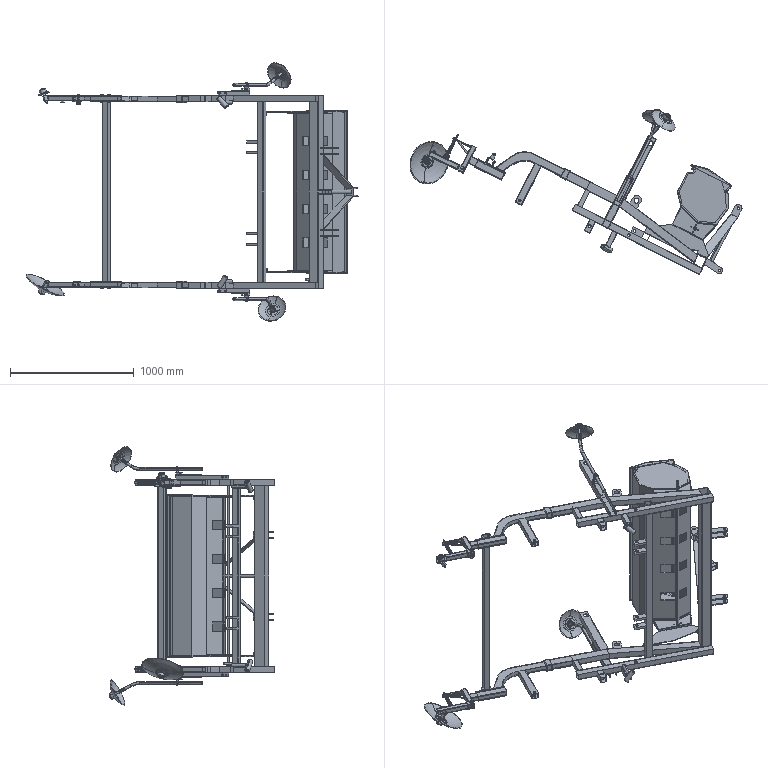Assembly | SolidWorks | mm | 102 component files | 111 solids | 2914 faces | box 2680.38 x 1339.53 x 2086.82 mm | volume 24526050 mm3 | plane 1099 | cylinder 917 | torus 468 | sphere 224 | cone 148 | spline 58 | commonest cylinder face diameters 20 x162 10 x114 8.5 x56 40 x50 8 x42 4 x40 12 x34 20.667 x32
Bill of materials:
AdjustmentEarPlate | 1 |  | U-shaped bent-sheet bracket: two parallel tapered flanges joined by a narrow web with rounded bends; each flange has a round hole near the web end.
Part24 | 2 |  | Combined profile: an open-ended thin-walled rectangular hollow tube with a round hollow tube of similar length lying along and joined to its top face.
Part26 | 2 |  | T-shaped part: a short thick-walled hollow cylinder with a smaller solid round rod sticking out at right angles from its side.
AttachedSoilDiskDiameter350 | 1 |  | Thin, shallow, concave dish-shaped disc with a central round hole and four smaller holes evenly spaced on a circle around it.
circlips for hole--type b gb | 4 |  | Flat split ring with a gap; the two ends form lugs that extend inward from the ring, each with a small round hole. The shape resembles an internal-style retaining ring.
circlips for shaft--type a large gb | 4 |  | Flat split ring with a narrow gap; the two ends form lugs that extend outward beyond the ring, each with a small round hole. The shape resembles an external-style retaining ring.
deep groove ball bearings gb | 8 |  | Ball-bearing-like ring assembly: an outer ring and an inner ring of equal width, with one row of spherical balls between them.
DustCover | 4 |  | Stepped annular ring: a wider, thin base flange with a smaller raised collar on top, a central through bore, and an open recess on the underside.
LargeAttachedSoilDiskAxis | 2 |  | Stepped cylindrical pin: a thin flat head, a long main shank, and a shorter reduced-diameter end section.
SoilDiskBearingHousing | 4 |  | Flanged sleeve: a hollow cylindrical boss on a thin circular flange that has four through holes evenly spaced around it.
AttachedSoilWheelVerticalAxis2 | 2 |  | T-shaped part: a short hollow cylindrical sleeve with a solid round rod sticking out at right angles from its side; the rod has a small cross hole near its free end.
FilmPressingSoilWheelBracket | 2 |  | T-shaped frame of thin-walled rectangular hollow tubes with a triangular gusset plate. The cross tube has a round hole, and a smaller telescoping-looking section with a hole extends from one end of a tube.
hex nuts with flange-fine pitch gb | 2 |  | Flanged hex nut-like body: hexagonal prism with a wider circular flange at one end and a plain central through-bore.
hexagon head bolts-full thread gb | 4 |  | Hex-head bolt-like part: hexagonal head on a plain cylindrical shank with a chamfered tip.
PressingFilmSoilPlateMovableFrame | 2 |  | Long arm with a rectangular cross-section: a cross-hole at one end, a forked (clevis-like) end with two parallel holed lugs at the other, and a pair of small parallel holed tabs sticking out from one side.
split pins | 2 |  | Split-pin-like part: two half-round legs side by side, joined by a looped eye at one end, with one leg longer than the other.
Spring3 | 2 |  | Helical coil spring made of round wire, with closely spaced end coils and evenly spaced open coils between them.
TieRod2 | 2 |  | Long cylindrical rod with a flat eye tab at one end and a circular collar near that end.
Part11 | 2 |  | Straight square or rectangular bar with a small holed tab sticking out sideways near one end.
Part5 | 2 |  | Short straight length of thin-walled rectangular tube, open at both ends.
Part5ConnectingSleeve | 2 |  | Short rectangular ring or sleeve with rounded outer edges, open through on one axis, with a raised rounded rib or seam across the faces.
Part6 | 2 |  | L-shaped frame made of two square or rectangular bars joined at roughly 90 degrees, with a through-hole near the free end of one arm.
Part7 | 2 |  | Straight length of thin-walled square or rectangular tube with open ends.
Part8 | 2 |  | Long slender square or rectangular tube with a single small round through-hole away from the ends.
PartFrameCorner | 2 |  | Welded-looking frame made of hollow rectangular tube: one long straight member with a smooth radiused bend at one end, plus a straight branch tube that joins it at an angle, forming a lambda/Y-like shape.
GB_T5781-2000[HexHeadBoltFullThreadGradeCM8_20] | 2 |  | Hex-head bolt-like part: a hexagonal head with a plain cylindrical shank coming out of one face. The shank has a chamfered free end, and there is a raised round collar/washer face between the head and the shank.
GB_T6174-2000[HexThinNutNoChamferM8] | 2 |  | Thin hexagonal nut-like part: a flat hex prism with one centred round through-hole, and chamfered corners on both faces.
Part10 | 1 |  | Straight length of hollow square tube with plain square-cut ends.
Part13 | 1 |  | Long hollow square tube with two pairs of thin parallel plate tabs sticking out from one side, one pair near each end. Each tab extends beyond the tube profile and has a round hole.
Part15 | 4 |  | Flat plate link with one rounded end that has a through hole; the plate widens toward the opposite, straight-cut end, which has a small corner chamfer.
Part17 | 1 |  | Thin flat plate with an irregular polygon outline and short bent flanges or lips along some edges, all turned to one side (downward in the side views).
Part18 | 1 |  | Thin flat plate with an irregular polygon outline and short flanges along some edges that point the opposite way from unnamed part (upward in the side views).
Part19 | 1 |  | Very slender solid round rod or pin with a constant diameter; the ends appear rounded or domed.
Part21 | 1 |  | Straight-cut spur gear with about 16 teeth, a central round bore and a cylindrical hub boss on one face.
Part28 | 2 |  | Short piece of hollow rectangular tube with open ends and one round through hole in a broad face.
Part40 | 1 |  | Straight length of hollow square tube with a relatively thick wall and plain ends.
PartThree | 4 |  | Flat plate with a constant thickness. One side has a wide rectangular notch that leaves two arms; the opposite side has two concave quarter-circle cutouts at its corners, leaving a narrower tongue.
AttachedSoilDisk | 2 |  | Thin dished (concave) circular disc with a flat central area that has a central round hole and four smaller holes evenly spaced around it.
AttachedSoilDiskAxis | 2 |  | Headed pin or bolt-like part: a thin, wide round head, a smooth cylindrical shank with a visible line around it partway along, and a grooved end section that looks threaded.
FilmBracketTube | 2 |  | Long, narrow formed sheet-metal channel (U- or hat-shaped cross-section), with a round hole near one end and a notch plus a bent hook or clip at the other end.
ScribingPlateFixedSleeve | 2 |  | Cylindrical sleeve that passes through a flat plate tab. The sleeve sticks out on both sides of the tab, and the tab has a stepped (L-shaped) top edge.
ScribingPlateMovableTube | 2 |  | Thin-walled round tube with one smooth bend near one end: a long straight leg and a short angled leg.
SeedBoxLidModification | 1 |  | Irregular polygonal plate with small notched tabs on one edge and a small hole pattern: a central hole with four smaller holes around it. The plate has a thicker region with raised edge walls or lips along part of its outline.
SeedBoxLidModificationOtherSide | 1 |  | Irregular polygonal flat plate with notched tabs on one edge, a central hole with four smaller holes around it, and one small hole near a tab. A region near one edge appears thicker.
SeedBoxModification | 1 |  | Long, open, roughly octagonal formed sheet-metal profile with hooked or stepped lips at both open edges, a row of rectangular slots along one face, and a small hole near one lip.
SeedBoxTopCover | 1 |  | Long, tapered, plate-like bracket or arm: a wide body that narrows toward a rounded lug with a round hole, plus a small stepped tab near the lug. One edge appears to have a narrow formed flange or lip.
TriangularHanger | 1 |  | V-shaped bracket made from two straight bars that meet at a vertex. At the vertex are a block with a hole and two parallel lugs with holes, in a clevis-like arrangement. The far ends of the bars are cut at an angle.
WeldedEarPlate | 1 |  | Flat tab: a rectangular block with one fully rounded end and one round through-hole centered on that rounded end. The opposite end is square.
WeldedPipe | 1 |  | Straight thin-walled round tube with plain square-cut ends.
Mates:
1. distance | Part15-4 face at (342.079, -1149.629, 1462.971) dir (0, 0, 1) | Part15-3 face at (342.079, -1149.629, 1502.971) dir (0, 0, -1)
2. coincident | AdjustmentEarPlate-1 face at (401.748, -1119.255, 1792.971) dir (0.4521, 0.892, 0) | WeldedPipe-1 edge at (366.069, -1101.171, 1812.971) dir (0.4521, 0.892, 0) r 16
3. concentric | TriangularHanger-1 edge at (550.526, -737.249, 1812.971) dir (0.4521, 0.892, 0) r 16 | WeldedPipe-1 edge at (551.43, -735.465, 1812.971) dir (0.4521, 0.892, 0) r 13
4. coincident | Part18-1 face at (350.003, -960.479, 1167.971) dir (0.4521, 0.892, 0) | SeedBoxAssemblyModified-1/SeedBoxLidModification-2 face at (47.001, -806.9, 1182.971) dir (-0.4521, -0.892, 0)
5. coincident | Part18-1 face at (298.812, -1061.476, 1162.971) dir (0, 0, -1) | SeedBoxAssemblyModified-1/SeedBoxLidModification-2 face at (240.361, -400.339, 1162.971) dir (0, 0, -1)
6. coincident | Part17-1 face at (45.644, -809.576, 2457.971) dir (-0.892, 0.4521, 0) | SeedBoxAssemblyModified-1/SeedBoxLidModificationOtherSide-1 face at (119.337, -664.185, 2442.971) dir (-0.892, 0.4521, 0)
7. coincident | SeedBoxAssemblyModified-1/SeedBoxLidModification-2 face at (214.293, -342.706, 1166.971) dir (0.4521, 0.892, 0) | SeedBoxTopCover-1 face at (196.453, -333.664, 1157.971) dir (-0.4521, -0.892, 0)
8. distance | SeedBoxAssemblyModified-1/SeedBoxModification-2 face at (526.481, -500.941, 2456.971) dir (0.892, -0.4521, 0) | SeedBoxTopCover-1 face at (526.481, -500.941, 1157.971) dir (0.892, -0.4521, 0)
9. concentric | SeedBoxTopCover-1 edge at (483.916, -540.681, 2467.971) dir (0, 0, 1) r 5 | GB_T5781-2000[HexHeadBoltFullThreadGradeCM8_20]-2 edge at (483.916, -540.681, 2448.971) dir (0, 0, 1) r 4
10. concentric | GB_T5781-2000[HexHeadBoltFullThreadGradeCM8_20]-1 edge at (483.792, -540.614, 1176.971) dir (0, 0, -1) r 4 | GB_T6174-2000[HexThinNutNoChamferM8]-1 edge at (483.792, -540.614, 1168.971) dir (0, 0, 1) r 4
11. concentric | GB_T5781-2000[HexHeadBoltFullThreadGradeCM8_20]-2 edge at (483.916, -540.681, 2448.971) dir (0, 0, 1) r 4 | GB_T6174-2000[HexThinNutNoChamferM8]-2 edge at (483.916, -540.681, 2456.971) dir (0, 0, 1) r 4
12. coincident | SeedBoxAssemblyModified-1/SeedBoxModification-2 face at (240.361, -400.339, 2456.971) dir (0, 0, -1) | GB_T6174-2000[HexThinNutNoChamferM8]-2 face at (477.416, -529.423, 2456.971) dir (0, 0, 1)
13. parallel | SeedBoxAssemblyModified-1/SeedBoxModification-2 face at (526.481, -500.941, 2456.971) dir (0.892, -0.4521, 0) | SeedBoxTopCover-1 face at (526.481, -500.941, 1157.971) dir (0.892, -0.4521, 0)
14. coincident | SeedBoxAssemblyModified-1/SeedBoxLidModification-2 face at (240.361, -400.339, 1162.971) dir (0, 0, -1) | SeedBoxTopCover-1 face at (466.915, -496.983, 1162.971) dir (0, 0, 1)
15. distance | GB_T6174-2000[HexThinNutNoChamferM8]-1 face at (477.292, -529.356, 1172.971) dir (0, 0, 1) | GB_T5781-2000[HexHeadBoltFullThreadGradeCM8_20]-1 face at (483.792, -540.614, 1177.971) dir (0, 0, 1)
16. distance | SeedBoxAssemblyModified-1/SeedBoxModification-2 face at (240.361, -400.339, 1168.971) dir (0, 0, 1) | GB_T6174-2000[HexThinNutNoChamferM8]-1 face at (477.292, -529.356, 1172.971) dir (0, 0, 1)
17. concentric | SeedBoxAssemblyModified-1/SeedBoxLidModification-2 edge at (483.792, -540.614, 1162.971) dir (0, 0, 1) r 4 | GB_T5781-2000[HexHeadBoltFullThreadGradeCM8_20]-1 edge at (483.792, -540.614, 1177.971) dir (0, 0, 1) r 3
18. concentric | GB_T5781-2000[HexHeadBoltFullThreadGradeCM8_20]-1 edge at (483.792, -540.614, 1176.971) dir (0, 0, -1) r 4 | GB_T6174-2000[HexThinNutNoChamferM8]-1 edge at (483.792, -540.614, 1172.971) dir (0, 0, 1) r 4
19. parallel | SeedBoxAssemblyModified-1/SeedBoxModification-2 face at (240.361, -400.339, 2456.971) dir (0, 0, -1) | GB_T6174-2000[HexThinNutNoChamferM8]-2 face at (477.416, -529.423, 2452.971) dir (0, 0, -1)
20. concentric | GB_T5781-2000[HexHeadBoltFullThreadGradeCM8_20]-2 edge at (483.916, -540.681, 2448.971) dir (0, 0, 1) r 4 | GB_T6174-2000[HexThinNutNoChamferM8]-2 edge at (483.916, -540.681, 2452.971) dir (0, 0, 1) r 4
21. distance | GB_T5781-2000[HexHeadBoltFullThreadGradeCM8_20]-2 face at (483.916, -540.681, 2447.971) dir (0, 0, -1) | GB_T6174-2000[HexThinNutNoChamferM8]-2 face at (477.416, -529.423, 2452.971) dir (0, 0, -1)
22. parallel | SeedBoxAssemblyModified-1/SeedBoxModification-2 face at (240.361, -400.339, 1168.971) dir (0, 0, 1) | GB_T5781-2000[HexHeadBoltFullThreadGradeCM8_20]-1 face at (483.792, -540.614, 1177.971) dir (0, 0, 1)
23. parallel | SeedBoxAssemblyModified-1/SeedBoxModification-2 face at (240.361, -400.339, 1168.971) dir (0, 0, 1) | GB_T5781-2000[HexHeadBoltFullThreadGradeCM8_20]-1 face at (483.792, -540.614, 1177.971) dir (0, 0, 1)
24. concentric | SeedBoxAssemblyModified-1/SeedBoxLidModificationOtherSide-1 edge at (231.081, -840.363, 2462.971) dir (0, 0, 1) r 13 | Part19-1 edge at (231.081, -840.363, 1045.971) dir (0, 0, 1) r 8.5
25. distance | Part19-1 face at (231.081, -840.363, 2582.971) dir (0, 0, 1) | SeedBoxAssemblyModified-1/SeedBoxLidModificationOtherSide-1 face at (240.361, -400.339, 2462.971) dir (0, 0, 1)
26. concentric | Part19-1 edge at (231.081, -840.363, 1045.971) dir (0, 0, 1) r 8.5 | Part21-2 edge at (231.081, -840.363, 1077.971) dir (0, 0, 1) r 16
27. distance | SeedBoxAssemblyModified-1/SeedBoxLidModification-2 face at (240.361, -400.339, 1162.971) dir (0, 0, -1) | Part21-2 face at (231.081, -840.363, 1097.971) dir (0, 0, -1)
28. coincident | Part17-1 face at (296.751, -933.488, 2457.971) dir (0.4521, 0.892, 0) | SeedBoxAssemblyModified-1/SeedBoxLidModificationOtherSide-1 face at (47.001, -806.9, 2442.971) dir (-0.4521, -0.892, 0)
29. coincident | Part17-1 face at (250.113, -1042.398, 2462.971) dir (0, 0, 1) | SeedBoxAssemblyModified-1/SeedBoxLidModificationOtherSide-1 face at (240.361, -400.339, 2462.971) dir (0, 0, 1)
30. coincident | FrameAssemblyDrawing11111-1/Part5-1 face at (-1544.877, -342.73, 1086.971) dir (-0.892, 0.4521, 0) | FrameAssemblyDrawing11111-Copy-1/Part5-1 face at (-1544.877, -342.73, 2590.971) dir (-0.892, 0.4521, 0)
31. parallel | FrameAssemblyDrawing11111-1/PartFrameCorner-1 face at (-1140.963, -396.106, 1080.971) dir (0, 0, 1) | FrameAssemblyDrawing11111-Copy-1/PartFrameCorner-1 face at (-1140.963, -396.106, 2544.971) dir (0, 0, -1)
32. coincident | FrameAssemblyDrawing11111-1/Part5-1 face at (-1543.521, -340.054, 1086.971) dir (0.4521, 0.892, 0) | PressingFilmSoilMechanism2-2/FilmPressingSoilWheelBracket-1 face at (-1329.449, -448.558, 1078.971) dir (-0.4521, -0.892, 0)
33. coincident | FrameAssemblyDrawing11111-1/Part5-1 face at (-1495.399, -380.35, 1083.971) dir (0, 0, -1) | PressingFilmSoilMechanism2-2/FilmPressingSoilWheelBracket-1 face at (-1327.189, -444.098, 1083.971) dir (0, 0, 1)
34. coincident | FrameAssemblyDrawing11111-1/Part5-1 face at (-1299.158, -388.796, 1086.971) dir (0.892, -0.4521, 0) | PressingFilmSoilMechanism2-2/FilmPressingSoilWheelBracket-1 face at (-1327.189, -444.098, 1048.971) dir (0.892, -0.4521, 0)
35. concentric | PressingFilmSoilMechanism2-2/AttachedSoilWheelVerticalAxis2-1 edge at (-1920.715, -303.338, 1046.651) dir (0.4522, -0.2133, 0.866) r 16 | AttachedSoilDiskDiameter350-2 edge at (-1930.212, -298.858, 1028.464) dir (-0.4522, 0.2133, -0.866) r 15
36. distance | AttachedSoilDiskDiameter350-2 face at (-1915.4, -246.677, 1037.046) dir (0.4522, -0.2133, 0.866) | PressingFilmSoilMechanism2-2/AttachedSoilWheelVerticalAxis2-1 face at (-1902.626, -311.87, 1081.292) dir (0.4522, -0.2133, 0.866)
37. coincident | FrameAssemblyDrawing11111-Copy-1/Part5-1 face at (-1543.521, -340.054, 2590.971) dir (0.4521, 0.892, 0) | FilmPressingSoilCoveringMechanism2Reverse-2/FilmPressingSoilWheelBracket-1 face at (-1329.449, -448.558, 2582.971) dir (-0.4521, -0.892, 0)
38. coincident | FrameAssemblyDrawing11111-Copy-1/Part5-1 face at (-1495.399, -380.35, 2587.971) dir (0, 0, -1) | FilmPressingSoilCoveringMechanism2Reverse-2/FilmPressingSoilWheelBracket-1 face at (-1327.189, -444.098, 2587.971) dir (0, 0, 1)
39. coincident | FrameAssemblyDrawing11111-Copy-1/Part5-1 face at (-1299.158, -388.796, 2590.971) dir (0.892, -0.4521, 0) | FilmPressingSoilCoveringMechanism2Reverse-2/FilmPressingSoilWheelBracket-1 face at (-1327.189, -444.098, 2552.971) dir (0.892, -0.4521, 0)
40. coincident | FrameAssemblyDrawing11111-Copy-1/Part5-1 face at (-1513.23, -280.292, 2590.971) dir (0.4521, 0.892, 0) | Part40-2 face at (-1406.194, -334.544, 1040.971) dir (-0.4521, -0.892, 0)
41. coincident | FrameAssemblyDrawing11111-Copy-1/Part5-1 face at (-1495.399, -380.35, 2590.971) dir (0, 0, 1) | Part40-2 face at (-1396.758, -291.07, 2590.971) dir (0, 0, 1)
42. distance | Part40-2 face at (-1450.793, -311.939, 1040.971) dir (-0.892, 0.4521, 0) | FrameAssemblyDrawing11111-Copy-1/Part5-1 face at (-1544.877, -342.73, 2590.971) dir (-0.892, 0.4521, 0)
43. distance | SeedBoxAssemblyModified-1/SeedBoxLidModification-2 face at (119.337, -664.185, 1182.971) dir (-0.892, 0.4521, 0) | Part18-1 face at (45.644, -809.576, 1182.971) dir (-0.892, 0.4521, 0)
44. coincident | FrameAssemblyDrawing11111-1/Part8-1 face at (-697.013, -707.415, 1035.971) dir (0, 0, -1) | Part10-1 face at (259.033, -1046.919, 1035.971) dir (0, 0, -1)
45. coincident | FrameAssemblyDrawing11111-1/Part8-1 face at (-733.735, -644.627, 1085.971) dir (0.4521, 0.892, 0) | Part10-1 face at (218.344, -1127.196, 1035.971) dir (-0.4521, -0.892, 0)
46. coincident | FrameAssemblyDrawing11111-1/Part11-2 face at (224.515, -1115.02, 1085.971) dir (0.892, -0.4521, 0) | Part10-1 face at (228.832, -1106.504, 1097.113) dir (-0.892, 0.4521, 0)
47. parallel | FrameAssemblyDrawing11111-Copy-1/Part8-1 face at (-697.013, -707.415, 2589.971) dir (0, 0, 1) | Part10-1 face at (259.033, -1046.919, 2589.971) dir (0, 0, 1)
48. coincident | Part17-1 face at (296.552, -1065.936, 2432.971) dir (-0.4521, -0.892, 0) | Part10-1 face at (259.033, -1046.919, 1035.971) dir (0.4521, 0.892, 0)
49. parallel | Part17-1 face at (250.113, -1042.398, 2462.971) dir (0, 0, 1) | FrameAssemblyDrawing11111-Copy-1/Part8-1 face at (-697.013, -707.415, 2589.971) dir (0, 0, 1)
50. coincident | Part17-1 face at (330.39, -1083.087, 2462.971) dir (0.892, -0.4521, 0) | Part10-1 face at (300.189, -1142.672, 1097.113) dir (0.892, -0.4521, 0)
51. distance | Part18-1 face at (298.812, -1061.476, 1162.971) dir (0, 0, -1) | FrameAssemblyDrawing11111-1/Part11-2 face at (-325.695, -673.671, 1085.971) dir (0, 0, 1)
52. parallel | Part17-1 face at (250.113, -1042.398, 2462.971) dir (0, 0, 1) | FrameAssemblyDrawing11111-Copy-1/Part11-2 face at (-325.695, -673.671, 2539.971) dir (0, 0, -1)
53. coincident | FrameAssemblyDrawing11111-Copy-1/Part8-1 face at (-697.013, -707.415, 2589.971) dir (0, 0, 1) | Part13-1 face at (-131.289, -893.926, 2589.971) dir (0, 0, 1)
54. coincident | FrameAssemblyDrawing11111-Copy-1/Part8-1 face at (-733.735, -644.627, 2589.971) dir (0.4521, 0.892, 0) | Part13-1 face at (-153.894, -938.524, 2589.971) dir (-0.4521, -0.892, 0)
55. coincident | Part17-1 face at (-174.531, -868.645, 2457.971) dir (-0.892, 0.4521, 0) | Part13-1 face at (-204.696, -928.158, 2528.83) dir (-0.892, 0.4521, 0)
56. parallel | Part17-1 face at (-129.933, -891.25, 2432.971) dir (0.892, -0.4521, 0) | Part13-1 face at (-160.098, -950.763, 2528.83) dir (0.892, -0.4521, 0)
57. coincident | FrameAssemblyDrawing11111-1/Part8-1 face at (-697.013, -707.415, 1035.971) dir (0, 0, -1) | Part13-1 face at (-131.289, -893.926, 1035.971) dir (0, 0, -1)
58. coincident | FrameAssemblyDrawing11111-1/Part8-1 face at (-733.735, -644.627, 1085.971) dir (0.4521, 0.892, 0) | Part13-1 face at (-153.894, -938.524, 2589.971) dir (-0.4521, -0.892, 0)
59. coincident | TriangularHanger-1 face at (259.033, -1046.919, 1512.971) dir (-0.4521, -0.892, 0) | Part10-1 face at (259.033, -1046.919, 1035.971) dir (0.4521, 0.892, 0)
60. distance | TriangularHanger-1 face at (259.033, -1046.919, 1452.971) dir (0, 0, -1) | Part10-1 face at (259.033, -1046.919, 1035.971) dir (0, 0, -1)
61. coincident | TriangularHanger-1 face at (334.007, -1075.951, 1337.971) dir (0.892, -0.4521, 0) | Part10-1 face at (300.189, -1142.672, 1097.113) dir (0.892, -0.4521, 0)
62. coincident | WeldedPipe-1 face at (366.069, -1101.171, 1812.971) dir (-0.4521, -0.892, 0) | Part10-1 face at (259.033, -1046.919, 1035.971) dir (0.4521, 0.892, 0)
63. coincident | AdjustmentEarPlate-1 face at (330.39, -1083.087, 1792.971) dir (-0.892, 0.4521, 0) | Part10-1 face at (300.189, -1142.672, 1097.113) dir (0.892, -0.4521, 0)
64. distance | AdjustmentEarPlate-1 face at (379.326, -1130.313, 1792.971) dir (0, 0, -1) | Part10-1 face at (259.033, -1046.919, 1035.971) dir (0, 0, -1)
65. distance | Part15-4 face at (342.079, -1149.629, 1452.971) dir (0, 0, -1) | Part10-1 face at (259.033, -1046.919, 1035.971) dir (0, 0, -1)
66. coincident | Part15-4 face at (305.946, -1131.315, 1462.971) dir (-0.892, 0.4521, 0) | Part10-1 face at (300.189, -1142.672, 1097.113) dir (0.892, -0.4521, 0)
67. coincident | Part15-4 face at (366.524, -1101.402, 1462.971) dir (0.4521, 0.892, 0) | Part10-1 face at (259.033, -1046.919, 1035.971) dir (0.4521, 0.892, 0)
68. coincident | Part15-3 face at (305.946, -1131.315, 1512.971) dir (-0.892, 0.4521, 0) | Part10-1 face at (300.189, -1142.672, 1097.113) dir (0.892, -0.4521, 0)
69. coincident | Part15-3 face at (366.524, -1101.402, 1512.971) dir (0.4521, 0.892, 0) | Part10-1 face at (259.033, -1046.919, 1035.971) dir (0.4521, 0.892, 0)
70. distance | Part15-2 face at (342.079, -1149.629, 2172.971) dir (0, 0, 1) | Part10-1 face at (259.033, -1046.919, 2589.971) dir (0, 0, 1)
71. coincident | Part15-2 face at (305.946, -1131.315, 2172.971) dir (-0.892, 0.4521, 0) | Part10-1 face at (300.189, -1142.672, 1097.113) dir (0.892, -0.4521, 0)
72. coincident | Part15-2 face at (366.524, -1101.402, 2172.971) dir (0.4521, 0.892, 0) | Part10-1 face at (259.033, -1046.919, 1035.971) dir (0.4521, 0.892, 0)
73. coincident | Part15-1 face at (305.946, -1131.315, 2122.971) dir (-0.892, 0.4521, 0) | Part10-1 face at (300.189, -1142.672, 1097.113) dir (0.892, -0.4521, 0)
74. coincident | Part15-1 face at (366.524, -1101.402, 2122.971) dir (0.4521, 0.892, 0) | Part10-1 face at (259.033, -1046.919, 1035.971) dir (0.4521, 0.892, 0)
75. distance | Part15-1 face at (342.079, -1149.629, 2122.971) dir (0, 0, 1) | Part15-2 face at (342.079, -1149.629, 2162.971) dir (0, 0, -1)
76. coincident | PartThree-2 face at (-1397.275, -339.065, 1040.971) dir (-0.4521, -0.892, 0) | FrameAssemblyDrawing11111-1/Part5-1 face at (-1513.23, -280.292, 1086.971) dir (0.4521, 0.892, 0)
77. coincident | PartThree-2 face at (-1404.056, -352.445, 1040.971) dir (0, 0, 1) | FrameAssemblyDrawing11111-1/Part5-1 face at (-1495.399, -380.35, 1040.971) dir (0, 0, -1)
78. coincident | PartThree-2 face at (-1404.942, -332.074, 1058.529) dir (-0.892, 0.4521, 0) | Part40-2 face at (-1406.194, -334.544, 1040.971) dir (0.892, -0.4521, 0)
79. coincident | PartThree-1 face at (-1459.712, -307.418, 1086.971) dir (-0.4521, -0.892, 0) | FrameAssemblyDrawing11111-1/Part5-1 face at (-1513.23, -280.292, 1086.971) dir (0.4521, 0.892, 0)
80. coincident | PartThree-1 face at (-1466.494, -320.798, 1086.971) dir (0, 0, -1) | FrameAssemblyDrawing11111-1/Part5-1 face at (-1495.399, -380.35, 1086.971) dir (0, 0, 1)
81. coincident | PartThree-1 face at (-1449.541, -309.469, 1069.414) dir (0.892, -0.4521, 0) | Part40-2 face at (-1450.793, -311.939, 1040.971) dir (-0.892, 0.4521, 0)
82. coincident | PartThree-3 face at (-1450.793, -311.939, 2544.971) dir (-0.4521, -0.892, 0) | FrameAssemblyDrawing11111-Copy-1/Part5-1 face at (-1513.23, -280.292, 2590.971) dir (0.4521, 0.892, 0)
83. coincident | PartThree-3 face at (-1457.574, -325.319, 2590.971) dir (0, 0, -1) | FrameAssemblyDrawing11111-Copy-1/Part5-1 face at (-1495.399, -380.35, 2590.971) dir (0, 0, 1)
84. coincident | PartThree-3 face at (-1449.541, -309.469, 2562.529) dir (0.892, -0.4521, 0) | Part40-2 face at (-1450.793, -311.939, 1040.971) dir (-0.892, 0.4521, 0)
85. coincident | PartThree-4 face at (-1406.194, -334.544, 2590.971) dir (-0.4521, -0.892, 0) | FrameAssemblyDrawing11111-Copy-1/Part5-1 face at (-1513.23, -280.292, 2590.971) dir (0.4521, 0.892, 0)
86. coincident | PartThree-4 face at (-1412.976, -347.924, 2544.971) dir (0, 0, 1) | FrameAssemblyDrawing11111-Copy-1/Part5-1 face at (-1495.399, -380.35, 2544.971) dir (0, 0, -1)
87. coincident | PartThree-4 face at (-1404.942, -332.074, 2573.414) dir (-0.892, 0.4521, 0) | Part40-2 face at (-1406.194, -334.544, 1040.971) dir (0.892, -0.4521, 0)
88. coincident | ScribingMechanismAssembly-2/FilmBracketTube-1 face at (-515.635, -816.834, 2624.971) dir (-0.4521, -0.892, 0) | FrameAssemblyDrawing11111-Copy-1/Part8-1 face at (-758.601, -693.686, 2589.971) dir (-0.4521, -0.892, 0)
89. coincident | ScribingMechanismAssembly-2/FilmBracketTube-1 face at (-312.19, -415.449, 2589.971) dir (0, 0, -1) | FrameAssemblyDrawing11111-Copy-1/Part8-1 face at (-697.013, -707.415, 2589.971) dir (0, 0, 1)
90. distance | ScribingMechanismAssembly-2/FilmBracketTube-1 face at (-263.132, -440.315, 2594.971) dir (0.892, -0.4521, 0) | Part10-1 face at (300.189, -1142.672, 1097.113) dir (0.892, -0.4521, 0)
91. coincident | ScribingMechanismAssembly-1/FilmBracketTube-1 face at (-471.037, -839.439, 1000.971) dir (-0.4521, -0.892, 0) | FrameAssemblyDrawing11111-1/Part8-1 face at (-758.601, -693.686, 1085.971) dir (-0.4521, -0.892, 0)
92. coincident | ScribingMechanismAssembly-1/FilmBracketTube-1 face at (-267.592, -438.054, 1035.971) dir (0, 0, 1) | FrameAssemblyDrawing11111-1/Part11-2 face at (-325.695, -673.671, 1035.971) dir (0, 0, -1)
93. distance | ScribingMechanismAssembly-1/FilmBracketTube-1 face at (-263.132, -440.315, 1030.971) dir (0.892, -0.4521, 0) | Part10-1 face at (300.189, -1142.672, 1097.113) dir (0.892, -0.4521, 0)
94. coincident | Assembly4-1/Part24-1 face at (-413.302, -868.703, 1089.08) dir (0.4521, 0.892, 0) | FrameAssemblyDrawing11111-1/Part8-1 face at (-758.601, -693.686, 1085.971) dir (-0.4521, -0.892, 0)
95. coincident | Assembly4-1/Part24-1 face at (-453.993, -993.824, 1035.971) dir (0, 0, -1) | FrameAssemblyDrawing11111-1/Part8-1 face at (-697.013, -707.415, 1035.971) dir (0, 0, -1)
96. distance | ScribingMechanismAssembly-1/FilmBracketTube-1 face at (-263.132, -440.315, 1030.971) dir (0.892, -0.4521, 0) | Assembly4-1/Part24-1 face at (-453.993, -993.824, 1075.971) dir (0.892, -0.4521, 0)
97. distance | AssemblyTillageDisc-1/Part24-1 face at (-453.993, -993.824, 2549.971) dir (0.892, -0.4521, 0) | ScribingMechanismAssembly-2/FilmBracketTube-1 face at (-263.132, -440.315, 2594.971) dir (0.892, -0.4521, 0)
98. coincident | AssemblyTillageDisc-1/Part24-1 face at (-490.156, -975.494, 2589.971) dir (0, 0, 1) | FrameAssemblyDrawing11111-Copy-1/Part8-1 face at (-697.013, -707.415, 2589.971) dir (0, 0, 1)
99. coincident | AssemblyTillageDisc-1/Part24-1 face at (-413.302, -868.703, 2536.863) dir (0.4521, 0.892, 0) | FrameAssemblyDrawing11111-Copy-1/Part8-1 face at (-758.601, -693.686, 2589.971) dir (-0.4521, -0.892, 0)
100. coincident | Part28-4 face at (-615.886, -766.022, 1085.971) dir (0.4521, 0.892, 0) | FrameAssemblyDrawing11111-1/Part8-1 face at (-758.601, -693.686, 1085.971) dir (-0.4521, -0.892, 0)
101. coincident | Part28-4 face at (-589.965, -818.378, 1035.971) dir (0, 0, -1) | FrameAssemblyDrawing11111-1/Part8-1 face at (-697.013, -707.415, 1035.971) dir (0, 0, -1)
102. coincident | Part28-3 face at (-615.886, -766.022, 2589.971) dir (0.4521, 0.892, 0) | FrameAssemblyDrawing11111-Copy-1/Part8-1 face at (-758.601, -693.686, 2589.971) dir (-0.4521, -0.892, 0)
103. coincident | Part28-3 face at (-589.965, -818.378, 2589.971) dir (0, 0, 1) | FrameAssemblyDrawing11111-Copy-1/Part8-1 face at (-697.013, -707.415, 2589.971) dir (0, 0, 1)
104. coincident | Part40-2 face at (-1383.589, -289.946, 1040.971) dir (0.4521, 0.892, 0) | WeldedEarPlate-5 face at (-1419.268, -271.862, 2550.971) dir (-0.4521, -0.892, 0)
105. distance | WeldedEarPlate-5 face at (-1390.065, -247.424, 2542.971) dir (0, 0, -1) | Part40-2 face at (-1396.758, -291.07, 2590.971) dir (0, 0, 1)
106. distance | Part40-2 face at (-1450.793, -311.939, 1040.971) dir (-0.892, 0.4521, 0) | WeldedEarPlate-5 face at (-1403.444, -240.643, 2550.971) dir (-0.892, 0.4521, 0)
107. distance | Part28-4 face at (-571.288, -788.627, 1085.971) dir (0.892, -0.4521, 0) | FrameAssemblyDrawing11111-1/Part8-1 face at (292.027, -1164.543, 1085.971) dir (0.892, -0.4521, 0)
108. distance | Part28-3 face at (-571.288, -788.627, 2589.971) dir (0.892, -0.4521, 0) | FrameAssemblyDrawing11111-Copy-1/Part8-1 face at (292.027, -1164.543, 2589.971) dir (0.892, -0.4521, 0)
109. concentric | Part24-1 face at (2.837, 36.367, 170) dir (0, -1, 0) r 15 | Part26-1 face at (2.837, -93.633, 170) dir (0, -1, 0) r 10
110. coincident | Part26-1 face at (2.837, -93.633, 170) dir (0, -1, 0) | Part24-1 face at (2.837, -93.633, 170) dir (0, -1, 0)
111. coincident | Part24-1 edge at (-24.743, 0.07636, 65) dir (0, 0, 1) r 10 | Part26-1 edge at (-24.743, 0.07636, 65) dir (0, 0, -1) r 10
112. concentric | FilmPressingSoilWheelBracket-1 face at (-20, -95, -170) dir (1, 0, 0) r 6 | PressingFilmSoilPlateMovableFrame-1 face at (25, -95, -170) dir (-1, 0, 0) r 6
113. coincident | FilmPressingSoilWheelBracket-1 face at (20, -120, -155) dir (1, 0, 0) | PressingFilmSoilPlateMovableFrame-1 face at (20, -115.929, -202.419) dir (-1, 0, 0)
114. concentric | PressingFilmSoilPlateMovableFrame-1 face at (0, 177.365, -442.841) dir (0, -0.9996, 0.02839) r 10 | AttachedSoilWheelVerticalAxis2-1 face at (0, -67.536, -435.887) dir (0, -0.9996, 0.02839) r 10
115. distance | AttachedSoilWheelVerticalAxis2-1 face at (0, -67.536, -435.887) dir (0, 0.9996, -0.02839) | PressingFilmSoilPlateMovableFrame-1 face at (-16, -83.24, -460.451) dir (0, 0.9996, -0.02839)
116. concentric | AttachedSoilWheelVerticalAxis2-1 face at (-18.794, -167.69, -439.886) dir (0.9397, 0.009709, 0.3419) r 10 | AttachedSoilDiskAssembly2-1/LargeAttachedSoilDiskAxis-1 face at (18.794, -167.302, -426.21) dir (-0.9397, -0.009709, -0.3419) r 10
117. coincident | AttachedSoilWheelVerticalAxis2-1 face at (18.794, -167.302, -426.21) dir (0.9397, 0.009709, 0.3419) | AttachedSoilDiskAssembly2-1/LargeAttachedSoilDiskAxis-1 face at (18.794, -167.302, -426.21) dir (0.9397, 0.009709, 0.3419)
118. angle | AttachedSoilWheelVerticalAxis2-1 face at (-18.794, -167.69, -439.886) dir (-0.9397, -0.009709, -0.3419) | PressingFilmSoilPlateMovableFrame-1 face at (20, -87.238, -460.337) dir (1, 0, 0)
119. concentric | AttachedSoilWheelVerticalAxis2-1 face at (-46.985, -79.017, -452.669) dir (0.9397, 0.009709, 0.3419) r 3 | split pins-1 face at (-9.794, -78.633, -439.138) dir (-0.9397, -0.009709, -0.3419) r 0.25
120. distance | split pins-1 face at (-12.613, -78.662, -440.164) dir (-0.9397, -0.009709, -0.3419) | AttachedSoilWheelVerticalAxis2-1 face at (0, -67.536, -435.887) dir (0, -0.9996, 0.02839) r 10
121. concentric | PressingFilmSoilPlateMovableFrame-1 face at (25, -95, -170) dir (-1, 0, 0) r 6 | hexagon head bolts-full thread gb-1 face at (10, -95, -170) dir (-1, 0, 0) r 4
122. coincident | PressingFilmSoilPlateMovableFrame-1 face at (-25, -114.424, -149.44) dir (-1, 0, 0) | hexagon head bolts-full thread gb-1 face at (-25, -95, -183) dir (1, 0, 0)
123. concentric | hexagon head bolts-full thread gb-1 face at (10, -95, -170) dir (-1, 0, 0) r 4 | hex nuts with flange-fine pitch gb-2 face at (25, -95, -170) dir (1, 0, 0) r 785.398
124. coincident | PressingFilmSoilPlateMovableFrame-1 face at (25, -115.929, -202.419) dir (1, 0, 0) | hex nuts with flange-fine pitch gb-2 face at (25, -110, -178.66) dir (-1, 0, 0)
125. concentric | PressingFilmSoilPlateMovableFrame-1 face at (-20, -62.057, -331) dir (1, 0, 0) r 5 | TieRod2-1 face at (27.5, -62.057, -331) dir (-1, 0, 0) r 5
126. distance | TieRod2-1 face at (2.5, -72.057, -321) dir (1, 0, 0) | PressingFilmSoilPlateMovableFrame-1 face at (5, -49.207, -318.86) dir (-1, 0, 0)
127. tangent | FilmPressingSoilWheelBracket-1 face at (0, -200, -330) dir (0, 1, 0) r 6 | TieRod2-1 face at (0, 137.943, -331) dir (0, -1, 0) r 5
128. concentric | TieRod2-1 face at (0, 137.943, -331) dir (0, -1, 0) r 5 | Spring3-1 sketch segment at (0, -22.057, -331) dir (0, 1, 0) r 10
129. coincident | TieRod2-1 face at (0, -22.057, -331) dir (0, 1, 0) | Spring3-1 face at (0, -22.057, -331) dir (0, -1, 0)
130. concentric | PressingFilmSoilPlateMovableFrame-1 face at (-20, -62.057, -331) dir (1, 0, 0) r 5 | hexagon head bolts-full thread gb-2 face at (25, -62.057, -331) dir (-1, 0, 0) r 4
131. coincident | PressingFilmSoilPlateMovableFrame-1 face at (-10, -49.207, -318.86) dir (-1, 0, 0) | hexagon head bolts-full thread gb-2 face at (-10, -62.057, -344) dir (1, 0, 0)
132. concentric | hexagon head bolts-full thread gb-2 face at (25, -62.057, -331) dir (-1, 0, 0) r 4 | hex nuts with flange-fine pitch gb-4 face at (10, -62.057, -331) dir (1, 0, 0) r 785.398
133. coincident | PressingFilmSoilPlateMovableFrame-1 face at (10, -49.207, -318.86) dir (1, 0, 0) | hex nuts with flange-fine pitch gb-4 face at (10, -77.057, -339.66) dir (-1, 0, 0)
134. concentric | SoilDiskBearingHousing-1 face at (72, 0, 0) dir (-1, 0, 0) r 23.5 | deep groove ball bearings gb-1 face at (59.289, 0, 0) dir (-1, 0, 0) r 13
135. coincident | SoilDiskBearingHousing-1 face at (72, 0, 0) dir (-1, 0, 0) | deep groove ball bearings gb-1 face at (72, 13, 0) dir (1, 0, 0)
136. concentric | SoilDiskBearingHousing-1 face at (72, 0, 0) dir (-1, 0, 0) r 23.5 | deep groove ball bearings gb-2 face at (51.289, 0, 0) dir (-1, 0, 0) r 13
137. coincident | deep groove ball bearings gb-1 face at (64, 13, 0) dir (-1, 0, 0) | deep groove ball bearings gb-2 face at (64, 13, 0) dir (1, 0, 0)
138. concentric | SoilDiskBearingHousing-1 face at (72, 0, 0) dir (-1, 0, 0) r 23.5 | circlips for hole--type b gb-1 face at (44, 0, 0) dir (-1, 0, 0) r 10.75
139. coincident | SoilDiskBearingHousing-1 face at (44, 0, 25.5) dir (-1, 0, 0) | circlips for hole--type b gb-1 face at (44, 0, 0) dir (1, 0, 0)
140. concentric | deep groove ball bearings gb-2 face at (53.029, 0, 0) dir (-1, 0, 0) r 5 | LargeAttachedSoilDiskAxis-1 face at (-21, 0, 0) dir (1, 0, 0) r 10
141. concentric | SoilDiskBearingHousing-1 face at (75, 0, 0) dir (-1, 0, 0) r 20 | DustCover-1 face at (77, 0, 0) dir (-1, 0, 0) r 20
142. coincident | SoilDiskBearingHousing-1 edge at (72, 0, 0) dir (-1, 0, 0) r 20 | DustCover-1 edge at (72, 0, 0) dir (1, 0, 0) r 20
143. concentric | LargeAttachedSoilDiskAxis-1 face at (-21, 0, 0) dir (1, 0, 0) r 10 | circlips for shaft--type a large gb-1 face at (43, 0, 0) dir (1, 0, 0) r 4.65
144. coincident | LargeAttachedSoilDiskAxis-1 face at (44, 2.228, -11.282) dir (-1, 0, 0) | circlips for shaft--type a large gb-1 face at (44, 0, 0) dir (1, 0, 0)
145. coincident | deep groove ball bearings gb-1 face at (72, 5, 0) dir (1, 0, 0) | LargeAttachedSoilDiskAxis-1 face at (72, 0, 0) dir (-1, 0, 0)
146. coincident | PartFrameCorner-1 face at (-461.187, -56.353, 753.41) dir (0, -1, 0) | Part5-1 face at (-612.187, -56.353, 759.41) dir (0, 1, 0)
147. distance | PartFrameCorner-1 edge at (-396.187, -56.353, 753.41) dir (0, 0, -1) | Part5-1 edge at (-372.187, -56.353, 759.41) dir (0, 0, -1)
148. coincident | PartFrameCorner-1 face at (-227.777, 8.647, 713.41) dir (0, 0, -1) | Part5-1 face at (-551.046, -137.54, 713.41) dir (0, 0, -1)
149. distance | Part5ConnectingSleeve-1 edge at (42.212, 186.082, 758.41) dir (0, 0, -1) | PartFrameCorner-1 edge at (-227.777, 183.647, 753.41) dir (0, 0, -1)
150. distance | PartFrameCorner-1 face at (-227.777, 8.647, 713.41) dir (0, 0, -1) | Part5ConnectingSleeve-1 face at (92.212, 191.082, 708.41) dir (0, 0, 1)
151. distance | Part5ConnectingSleeve-1 face at (92.212, 116.082, 703.41) dir (0, 1, 0) | PartFrameCorner-1 face at (-194.191, 118.515, 753.41) dir (0, -1, 0)
152. distance | PartFrameCorner-1 face at (-227.777, 8.647, 713.41) dir (0, 0, -1) | Part6-1 face at (114.746, 121.183, 710.41) dir (0, 0, 1)
153. distance | PartFrameCorner-1 face at (-227.777, 183.647, 753.41) dir (0, 1, 0) | Part6-1 face at (47.813, 184.082, 758.41) dir (0, -1, 0)
154. distance | Part6-1 face at (47.813, 186.082, 758.41) dir (-1, 0, 0) | Part5-1 face at (-372.187, -56.353, 759.41) dir (1, 0, 0)
155. distance | Part7-3 face at (267.813, 116.082, 758.41) dir (0, 0, 1) | Part6-1 face at (114.746, 121.183, 758.41) dir (0, 0, 1)
156. perpendicular | Part6-1 face at (47.813, 116.082, 758.41) dir (0, -1, 0) | Part7-3 face at (307.813, -78.46, 797.209) dir (1, 0, 0)
157. distance | Part7-3 face at (307.813, -78.46, 797.209) dir (1, 0, 0) | Part6-1 face at (577.813, 186.082, 758.41) dir (1, 0, 0)
158. distance | Part7-3 face at (267.813, -28.918, 708.41) dir (0, -1, 0) | Part6-1 face at (47.813, 116.082, 758.41) dir (0, -1, 0)
159. distance | Part7-3 face at (267.813, -78.46, 797.209) dir (-1, 0, 0) | Part8-1 face at (247.813, -28.918, 758.41) dir (-1, 0, 0)
160. distance | Part8-1 face at (247.813, -28.918, 758.41) dir (0, 1, 0) | Part7-3 face at (267.813, -28.918, 708.41) dir (0, -1, 0)
161. coincident | Part7-3 face at (267.813, 116.082, 708.41) dir (0, 0, -1) | Part8-1 face at (308.954, -68.32, 708.41) dir (0, 0, -1)
162. coincident | Part7-3 face at (267.813, 116.082, 708.41) dir (0, 0, -1) | Part8-1 face at (308.954, -68.32, 708.41) dir (0, 0, -1)
163. coincident | Part6-1 face at (114.746, 121.183, 708.41) dir (0, 0, -1) | Part11-2 face at (624.902, 129.651, 708.41) dir (0, 0, -1)
164. coincident | Part6-1 face at (47.813, 186.082, 758.41) dir (0, 1, 0) | Part11-2 edge at (577.813, 186.082, 758.41) dir (0, 0, -1)
165. coincident | Part6-1 edge at (577.813, 116.082, 708.41) dir (0, 1, 0) | Part11-2 edge at (577.813, 186.082, 708.41) dir (0, -1, 0)
166. coincident | PartFrameCorner-1 face at (-461.187, -56.353, 753.41) dir (0, -1, 0) | Part5-1 face at (-612.187, -56.353, 759.41) dir (0, 1, 0)
167. distance | PartFrameCorner-1 edge at (-396.187, -56.353, 753.41) dir (0, 0, -1) | Part5-1 edge at (-372.187, -56.353, 759.41) dir (0, 0, -1)
168. coincident | PartFrameCorner-1 face at (-227.777, 8.647, 713.41) dir (0, 0, -1) | Part5-1 face at (-551.046, -137.54, 713.41) dir (0, 0, -1)
169. distance | Part5ConnectingSleeve-1 edge at (42.212, 186.082, 758.41) dir (0, 0, -1) | PartFrameCorner-1 edge at (-227.777, 183.647, 753.41) dir (0, 0, -1)
170. distance | PartFrameCorner-1 face at (-227.777, 8.647, 713.41) dir (0, 0, -1) | Part5ConnectingSleeve-1 face at (92.212, 191.082, 708.41) dir (0, 0, 1)
171. distance | Part5ConnectingSleeve-1 face at (92.212, 116.082, 703.41) dir (0, 1, 0) | PartFrameCorner-1 face at (-194.191, 118.515, 753.41) dir (0, -1, 0)
172. distance | PartFrameCorner-1 face at (-227.777, 8.647, 713.41) dir (0, 0, -1) | Part6-1 face at (114.746, 121.183, 710.41) dir (0, 0, 1)
173. distance | PartFrameCorner-1 face at (-227.777, 183.647, 753.41) dir (0, 1, 0) | Part6-1 face at (47.813, 184.082, 758.41) dir (0, -1, 0)
174. distance | Part6-1 face at (47.813, 186.082, 758.41) dir (-1, 0, 0) | Part5-1 face at (-372.187, -56.353, 759.41) dir (1, 0, 0)
175. distance | Part7-3 face at (267.813, 116.082, 758.41) dir (0, 0, 1) | Part6-1 face at (114.746, 121.183, 758.41) dir (0, 0, 1)
176. perpendicular | Part6-1 face at (47.813, 116.082, 758.41) dir (0, -1, 0) | Part7-3 face at (307.813, -78.46, 797.209) dir (1, 0, 0)
177. distance | Part7-3 face at (307.813, -78.46, 797.209) dir (1, 0, 0) | Part6-1 face at (577.813, 186.082, 758.41) dir (1, 0, 0)
178. distance | Part7-3 face at (267.813, -28.918, 708.41) dir (0, -1, 0) | Part6-1 face at (47.813, 116.082, 758.41) dir (0, -1, 0)
179. distance | Part7-3 face at (267.813, -78.46, 797.209) dir (-1, 0, 0) | Part8-1 face at (247.813, -28.918, 758.41) dir (-1, 0, 0)
180. distance | Part8-1 face at (247.813, -28.918, 758.41) dir (0, 1, 0) | Part7-3 face at (267.813, -28.918, 708.41) dir (0, -1, 0)
181. coincident | Part7-3 face at (267.813, 116.082, 708.41) dir (0, 0, -1) | Part8-1 face at (308.954, -68.32, 708.41) dir (0, 0, -1)
182. coincident | Part7-3 face at (267.813, 116.082, 708.41) dir (0, 0, -1) | Part8-1 face at (308.954, -68.32, 708.41) dir (0, 0, -1)
183. coincident | Part6-1 face at (114.746, 121.183, 708.41) dir (0, 0, -1) | Part11-2 face at (624.902, 129.651, 708.41) dir (0, 0, -1)
184. coincident | Part6-1 face at (47.813, 186.082, 758.41) dir (0, 1, 0) | Part11-2 edge at (577.813, 186.082, 758.41) dir (0, 0, -1)
185. coincident | Part6-1 edge at (577.813, 116.082, 708.41) dir (0, 1, 0) | Part11-2 edge at (577.813, 186.082, 708.41) dir (0, -1, 0)
186. concentric | FilmPressingSoilWheelBracket-1 face at (-20, -95, -170) dir (1, 0, 0) r 6 | PressingFilmSoilPlateMovableFrame-1 face at (25, -95, -170) dir (-1, 0, 0) r 6
187. coincident | FilmPressingSoilWheelBracket-1 face at (20, -120, -155) dir (1, 0, 0) | PressingFilmSoilPlateMovableFrame-1 face at (20, -115.929, -202.419) dir (-1, 0, 0)
188. concentric | PressingFilmSoilPlateMovableFrame-1 face at (0, 177.365, -442.841) dir (0, -0.9996, 0.02839) r 10 | AttachedSoilWheelVerticalAxis2-1 face at (0, -67.536, -435.887) dir (0, -0.9996, 0.02839) r 10
189. distance | AttachedSoilWheelVerticalAxis2-1 face at (0, -67.536, -435.887) dir (0, 0.9996, -0.02839) | PressingFilmSoilPlateMovableFrame-1 face at (-16, -83.24, -460.451) dir (0, 0.9996, -0.02839)
190. concentric | AttachedSoilWheelVerticalAxis2-1 face at (17.321, -167.78, -443.044) dir (-0.866, 0.01419, 0.4998) r 10 | AttachedSoilDiskAssembly2-1/LargeAttachedSoilDiskAxis-1 face at (-17.321, -167.212, -423.052) dir (0.866, -0.01419, -0.4998) r 10
191. coincident | AttachedSoilWheelVerticalAxis2-1 face at (-17.321, -167.212, -423.052) dir (-0.866, 0.01419, 0.4998) | AttachedSoilDiskAssembly2-1/LargeAttachedSoilDiskAxis-1 face at (-17.321, -167.212, -423.052) dir (-0.866, 0.01419, 0.4998)
192. angle | AttachedSoilWheelVerticalAxis2-1 face at (17.321, -167.78, -443.044) dir (0.866, -0.01419, -0.4998) | PressingFilmSoilPlateMovableFrame-1 face at (20, -87.238, -460.337) dir (1, 0, 0)
193. concentric | AttachedSoilWheelVerticalAxis2-1 face at (43.301, -79.242, -460.564) dir (-0.866, 0.01419, 0.4998) r 3 | split pins-1 face at (9.026, -78.68, -440.784) dir (0.866, -0.01419, -0.4998) r 0.25
194. distance | split pins-1 face at (11.625, -78.722, -442.283) dir (0.866, -0.01419, -0.4998) | AttachedSoilWheelVerticalAxis2-1 face at (0, -67.536, -435.887) dir (0, -0.9996, 0.02839) r 10
195. concentric | PressingFilmSoilPlateMovableFrame-1 face at (25, -95, -170) dir (-1, 0, 0) r 6 | hexagon head bolts-full thread gb-1 face at (10, -95, -170) dir (-1, 0, 0) r 4
196. coincident | PressingFilmSoilPlateMovableFrame-1 face at (-25, -114.424, -149.44) dir (-1, 0, 0) | hexagon head bolts-full thread gb-1 face at (-25, -95, -183) dir (1, 0, 0)
197. concentric | PressingFilmSoilPlateMovableFrame-1 face at (-20, -62.057, -331) dir (1, 0, 0) r 5 | TieRod2-1 face at (27.5, -62.057, -331) dir (-1, 0, 0) r 5
198. distance | TieRod2-1 face at (2.5, -72.057, -321) dir (1, 0, 0) | PressingFilmSoilPlateMovableFrame-1 face at (5, -49.207, -318.86) dir (-1, 0, 0)
199. tangent | FilmPressingSoilWheelBracket-1 face at (0, -200, -330) dir (0, 1, 0) r 6 | TieRod2-1 face at (0, 137.943, -331) dir (0, -1, 0) r 5
200. concentric | TieRod2-1 face at (0, 137.943, -331) dir (0, -1, 0) r 5 | Spring3-1 sketch segment at (0, -22.057, -331) dir (0, 1, 0) r 10
201. coincident | TieRod2-1 face at (0, -22.057, -331) dir (0, 1, 0) | Spring3-1 face at (0, -22.057, -331) dir (0, -1, 0)
202. concentric | PressingFilmSoilPlateMovableFrame-1 face at (-20, -62.057, -331) dir (1, 0, 0) r 5 | hexagon head bolts-full thread gb-2 face at (25, -62.057, -331) dir (-1, 0, 0) r 4
203. coincident | PressingFilmSoilPlateMovableFrame-1 face at (-10, -49.207, -318.86) dir (-1, 0, 0) | hexagon head bolts-full thread gb-2 face at (-10, -62.057, -344) dir (1, 0, 0)
204. concentric | ScribingPlateMovableTube-1 face at (67, 564.808, 0) dir (0, -1, 0) r 12 | ScribingPlateFixedSleeve-1 face at (67, 243, 0) dir (0, -1, 0) r 15
205. coincident | FilmBracketTube-1 edge at (37, 225, 15) dir (0, 0, 1) | ScribingPlateFixedSleeve-1 face at (37, 205, 20) dir (1, 0, 0)
206. coincident | FilmBracketTube-1 edge at (40, 225, 25) dir (0, 0, -1) | ScribingPlateFixedSleeve-1 face at (37, 225, 20) dir (0, -1, 0)
207. concentric | ScribingPlateMovableTube-1 face at (85.495, 639.808, -7.861) dir (0.4602, 0.866, -0.1956) r 10 | AttachedSoilDiskAssembly-1/AttachedSoilDiskAxis-1 face at (113.016, 691.603, -19.557) dir (0.4602, 0.866, -0.1956) r 10
208. distance | AttachedSoilDiskAssembly-1/AttachedSoilDiskAxis-1 face at (113.016, 691.603, -19.557) dir (-0.4602, -0.866, 0.1956) | ScribingPlateMovableTube-1 face at (136.025, 734.904, -29.336) dir (0.4602, 0.866, -0.1956)
209. distance | FilmBracketTube-1 face at (25, 195, 27) dir (0, 0, -1) | ScribingPlateFixedSleeve-1 face at (37, 205, 20) dir (0, 0, 1)
210. coincident | FilmBracketTube-1 face at (37, 195, -25) dir (-1, 0, 0) | ScribingPlateFixedSleeve-1 face at (37, 205, 20) dir (1, 0, 0)
211. distance | ScribingPlateMovableTube-1 face at (67, 5, 0) dir (0, -1, 0) | FilmBracketTube-1 face at (15, -225, 25) dir (0, -1, 0)
212. concentric | SoilDiskBearingHousing-1 face at (62, 0, 0) dir (-1, 0, 0) r 23.5 | deep groove ball bearings gb-1 face at (49.289, 0, 0) dir (-1, 0, 0) r 13
213. coincident | SoilDiskBearingHousing-1 face at (62, 0, 0) dir (-1, 0, 0) | deep groove ball bearings gb-1 face at (62, 13, 0) dir (1, 0, 0)
214. concentric | SoilDiskBearingHousing-1 face at (62, 0, 0) dir (-1, 0, 0) r 23.5 | deep groove ball bearings gb-2 face at (41.289, 0, 0) dir (-1, 0, 0) r 13
215. coincident | deep groove ball bearings gb-1 face at (54, 13, 0) dir (-1, 0, 0) | deep groove ball bearings gb-2 face at (54, 13, 0) dir (1, 0, 0)
216. concentric | SoilDiskBearingHousing-1 face at (62, 0, 0) dir (-1, 0, 0) r 23.5 | circlips for hole--type b gb-1 face at (34, 0, 0) dir (-1, 0, 0) r 10.75
217. coincident | SoilDiskBearingHousing-1 face at (34, 0, 25.5) dir (-1, 0, 0) | circlips for hole--type b gb-1 face at (34, 0, 0) dir (1, 0, 0)
218. concentric | deep groove ball bearings gb-2 face at (43.029, 0, 0) dir (-1, 0, 0) r 5 | AttachedSoilDiskAxis-1 face at (-68, 0, 0) dir (1, 0, 0) r 10
219. concentric | AttachedSoilDisk-1 face at (20, 0, 0) dir (1, 0, 0) r 15 | SoilDiskBearingHousing-1 face at (65, 0, 0) dir (-1, 0, 0) r 27.5
220. concentric | AttachedSoilDisk-1 face at (20, 36, 0) dir (1, 0, 0) r 4.25 | SoilDiskBearingHousing-1 face at (30, 36, 0) dir (1, 0, 0) r 4.25
221. coincident | AttachedSoilDisk-1 face at (30, 60, 0) dir (1, 0, 0) | SoilDiskBearingHousing-1 face at (30, 0, 0) dir (-1, 0, 0)
222. concentric | SoilDiskBearingHousing-1 face at (65, 0, 0) dir (-1, 0, 0) r 20 | DustCover-1 face at (67, 0, 0) dir (-1, 0, 0) r 20
223. coincident | SoilDiskBearingHousing-1 edge at (62, 0, 0) dir (-1, 0, 0) r 20 | DustCover-1 edge at (62, 0, 0) dir (1, 0, 0) r 20
224. concentric | AttachedSoilDiskAxis-1 face at (-68, 0, 0) dir (1, 0, 0) r 10 | circlips for shaft--type a large gb-1 face at (33, 0, 0) dir (1, 0, 0) r 4.65
225. coincident | AttachedSoilDiskAxis-1 face at (34, 2.228, -11.282) dir (-1, 0, 0) | circlips for shaft--type a large gb-1 face at (34, 0, 0) dir (1, 0, 0)
226. coincident | deep groove ball bearings gb-1 face at (62, 5, 0) dir (1, 0, 0) | AttachedSoilDiskAxis-1 face at (62, 0, 0) dir (-1, 0, 0)
227. coincident | SeedBoxModification-2 face at (-177.323, 326.969, 358.601) dir (0, 0, -1) | SeedBoxLidModification-2 face at (-177.323, 326.969, 358.601) dir (0, 0, 1)
228. coincident | SeedBoxModification-2 face at (-226.631, 366.59, 1648.601) dir (0, 1, 0) | SeedBoxLidModification-2 face at (-226.631, 366.59, 358.601) dir (0, 1, 0)
229. coincident | SeedBoxModification-2 face at (-226.631, 366.59, 1648.601) dir (-1, 0, 0) | SeedBoxLidModification-2 face at (-226.631, 366.59, 358.601) dir (-1, 0, 0)
230. coincident | SeedBoxModification-2 face at (-177.323, 326.969, 1650.601) dir (0, 0, 1) | SeedBoxLidModificationOtherSide-1 face at (-177.323, 326.969, 1650.601) dir (0, 0, -1)
231. coincident | SeedBoxModification-2 face at (-226.631, 366.59, 1648.601) dir (0, 1, 0) | SeedBoxLidModificationOtherSide-1 face at (-226.631, 366.59, 1650.601) dir (0, 1, 0)
232. coincident | SeedBoxModification-2 face at (-226.631, 366.59, 1648.601) dir (-1, 0, 0) | SeedBoxLidModificationOtherSide-1 face at (-226.631, 366.59, 1650.601) dir (-1, 0, 0)